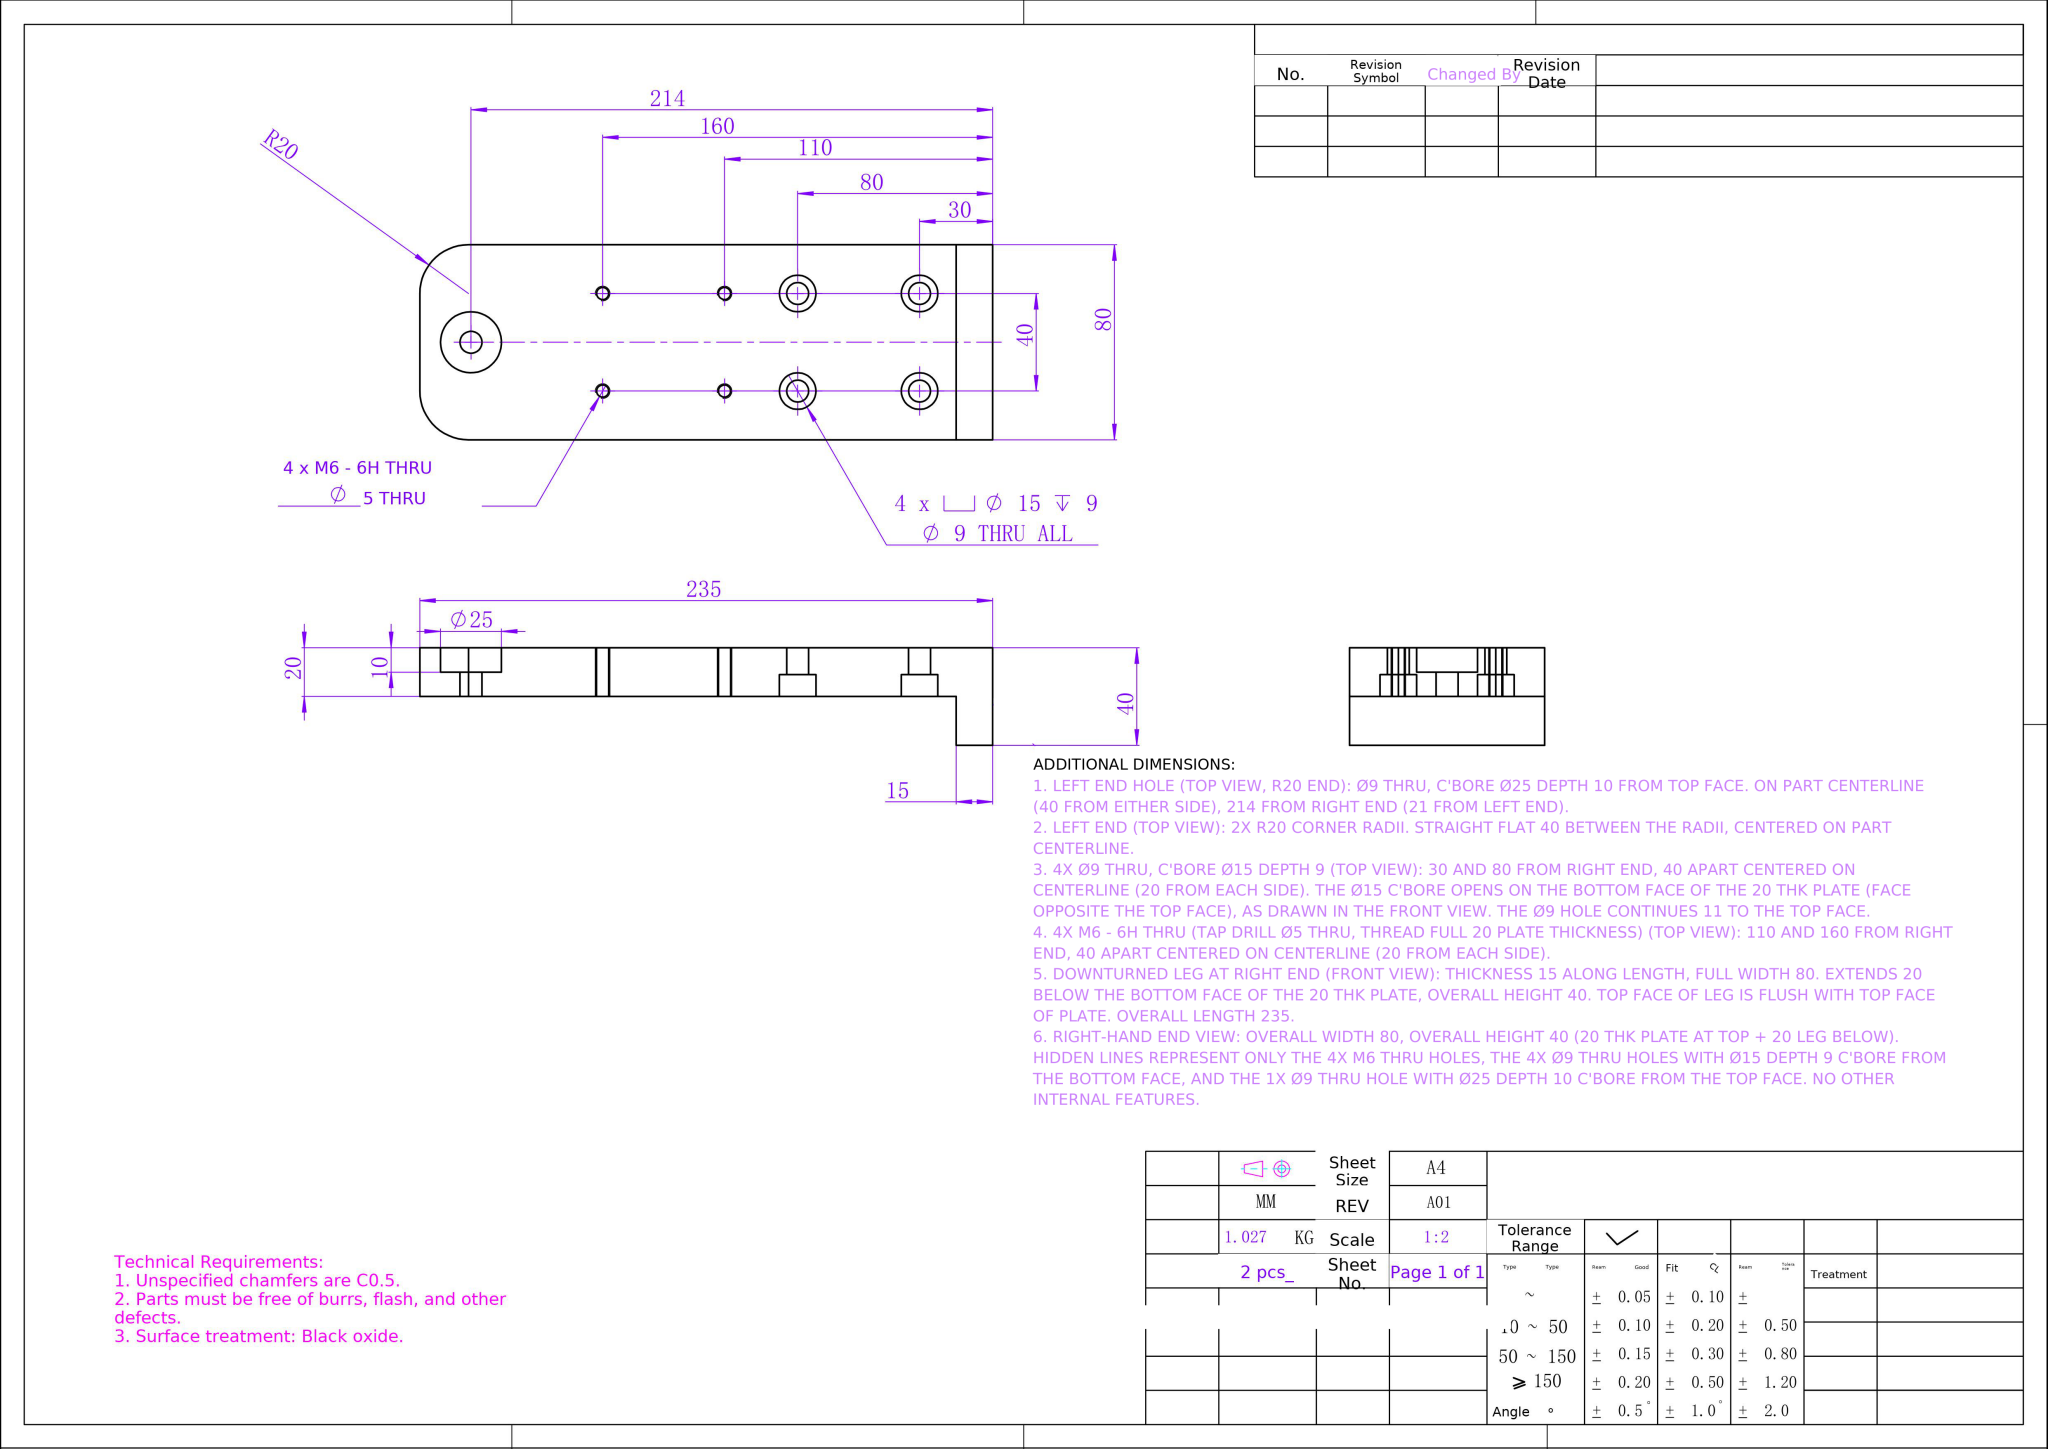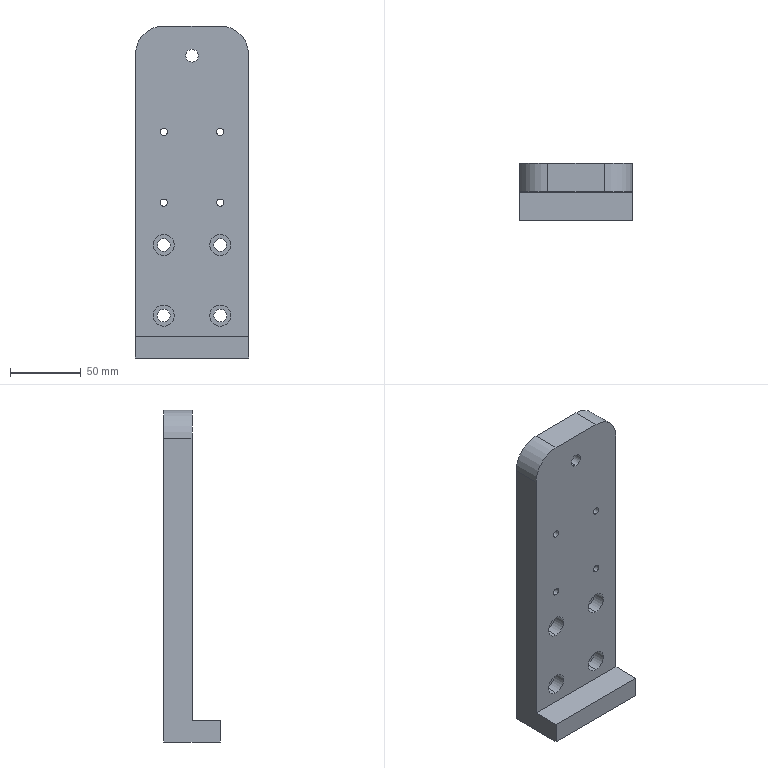Part | NX | mm | 1 solid | 43 faces | box 80 x 40 x 235 mm | volume 380290 mm3 | cylinder 30 | plane 13 | commonest cylinder face diameters 9 x10 5 x8 15 x8 25 x2 40 x2